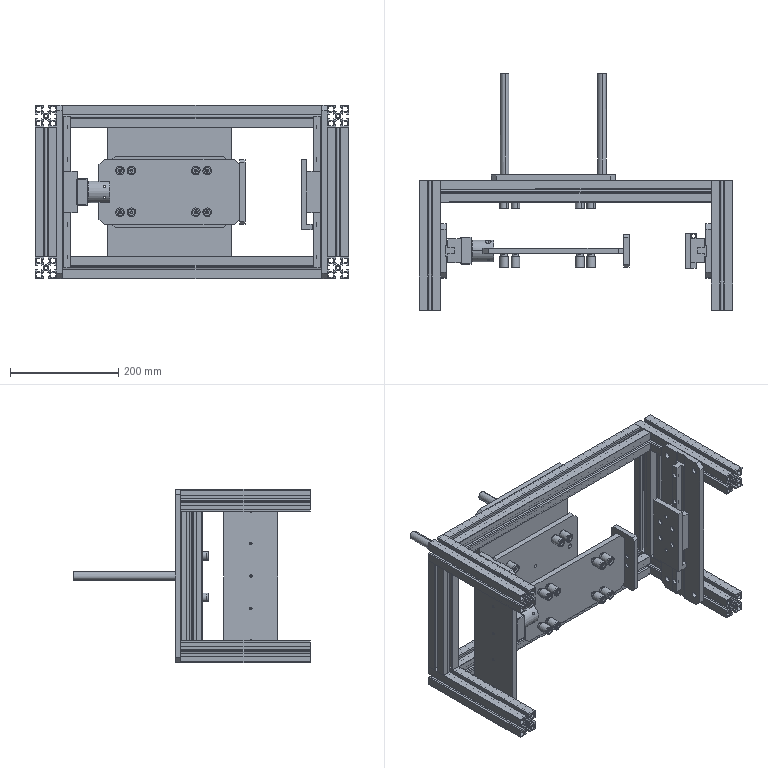Assembly | SolidWorks | mm | 41 component files | 41 solids | 1605 faces | box 580.04 x 437.8 x 320 mm | volume 3969042 mm3 | plane 981 | cylinder 594 | cone 30 | commonest cylinder face diameters 12 x96 5 x66 5.5 x44 16 x40 10 x40 4.2 x40 10.5 x40 5.3 x32
Bill of materials:
AdjustmentCylinderFixingPlate | 1 |  | Flat rectangular plate with four chamfered corners, one large central through-hole, and four small through-holes, one near each corner.
AdsorptionPlate | 1 |  | Thin, elongated rectangular plate with chamfered corners and eight through-holes in four pairs near the corners, plus two smaller holes near one short edge.
AdsorptionRelease | 1 |  | Thin rectangular plate with chamfered corners, eight larger through-holes in four pairs near the corners, and three smaller holes along the horizontal centerline (one at the center, one near each short edge).
AluminumProfile504 | 2 | 6061 Alloy | Long, straight prismatic extrusion with a square outer cross-section, an undercut slot centered on each of the four sides, hollow corner chambers, and a round central bore joined to the corners by diagonal webs.
Bearing6902 | 1 |  | Thick annular ring (flat washer- or spacer-like): a short hollow cylinder with a concentric through-bore and flat parallel faces.
GuideRailHGH-20CA-340 | 2 |  | Long, slender bar with a T-shaped cross-section (wide flange plus a narrower stem) and five evenly spaced small holes along its length.
GuideRod | 2 | AISI 304 | Long, straight, thick-walled round tube (hollow cylinder) with plain ends.
HGH20CASlider | 2 |  | Rectangular block with a full-height rectangular slot cut into one side, giving a C-shaped top profile, and four small holes in a rectangular pattern on one large face.
MainRotatingPlate | 1 |  | Moderately thick rectangular plate with chamfered corners and four small through-holes in a 2x2 pattern, placed off-center toward one long edge.
Profile240 | 6 | 6061 Alloy | Short length of square prismatic extrusion with an undercut slot on each side, hollow corner chambers, and a central round bore joined by diagonal webs.
RotationAxis | 1 |  | Cylindrical fork/clevis-like body: a large cylinder with a rectangular slot across one end that leaves two tines, cross-holes through the tines, and two stepped smaller-diameter coaxial bosses at the opposite end.
SidePlate | 2 |  | Elongated flat plate with chamfered corners, four corner holes, a centerline row of five small holes, and a stepped or recessed region on one face.
SlidingPlate | 1 |  | Square, fairly thick block with chamfered outer edges, a large central through bore, and four smaller through holes, one near each corner.
SwingCylinderMountingPlate | 1 |  | L-shaped bracket: a tall rectangular plate with a short perpendicular foot along its bottom edge. The plate has six through holes and the foot has one larger hole.
SuctionPositioning | 16 | AISI 304 | Stepped hollow cylinder: a larger-diameter section and a smaller-diameter section on one axis, with an axial bore all the way through and one radial cross hole through the smaller section.
UpperAndLowerCylinderMountingPlate | 1 |  | Thin, flat rectangular plate with chamfered corners. It has four elongated slots, one large central hole, two smaller holes to either side, and small holes clustered around each of these three holes.
Mates:
1. coincident | assembly face at (2922.223, 3603.91, 956.241) dir (0.0001552, -1, 0) | assembly face at (1637.199, 3603.71, 939.241) dir (-0.0001552, 1, 0)
2. distance | assembly face at (2922.22, 3618.61, 959.241) dir (0, 0, 1) | assembly face at (1502.198, 3608.689, 999.241) dir (0, 0, -1)
3. coincident | assembly face at (-641.795, 3680.91, 1199.241) dir (0, 0, -1) | assembly face at (1579.721, 3703.352, 1199.241) dir (0, 0, 1)
4. concentric | assembly face at (1554.723, 3703.361, 1192.741) dir (0, 0, -1) r 5.5 | assembly face at (1554.723, 3703.361, 965.741) dir (0, 0, 1) r 5.5
5. coincident | assembly face at (2922.211, 3680.91, 959.241) dir (0, 0, 1) | assembly face at (1529.723, 3703.357, 959.241) dir (0, 0, -1)
6. width | AdsorptionPlate-1 face at (1702.163, 3838.72, 1079.241) dir (-0.0001552, 1, 0) | AdsorptionPlate-1 face at (1702.164, 3828.72, 1079.241) dir (0.0001552, -1, 0) | MainRotatingPlate-1 face at (1832.159, 3863.74, 1019.241) dir (-0.0001552, 1, 0) | MainRotatingPlate-1 face at (1832.168, 3803.74, 1019.241) dir (0.0001552, -1, 0)
7. coincident | MainRotatingPlate-1 face at (1832.163, 3833.74, 1079.241) dir (-1, -0.0001552, 0) | AdsorptionPlate-1 face at (1832.163, 3838.74, 1011.741) dir (1, 0.0001552, 0)
8. width | AdsorptionPlate-1 face at (1832.163, 3838.74, 1019.241) dir (0, 0, -1) | AdsorptionPlate-1 face at (1832.163, 3838.74, 1139.241) dir (0, 0, 1) | MainRotatingPlate-1 face at (1832.159, 3863.74, 1139.241) dir (0, 0, 1) | MainRotatingPlate-1 face at (1832.159, 3863.74, 1019.241) dir (0, 0, -1)
9. coincident | AdsorptionPlate-1 face at (1702.163, 3838.72, 1079.241) dir (-0.0001552, 1, 0) | UltrasonicProductSuction-1/SuctionPositioning-1 face at (1772.163, 3838.731, 1041.741) dir (-0.0001552, 1, 0)
10. concentric | AdsorptionPlate-1 face at (1772.163, 3838.731, 1041.741) dir (-0.0001552, 1, 0) r 6 | UltrasonicProductSuction-1/SuctionPositioning-1 face at (1772.166, 3813.731, 1041.741) dir (-0.0001552, 1, 0) r 6
11. concentric | AdsorptionPlate-1 face at (1751.163, 3838.728, 1041.741) dir (-0.0001552, 1, 0) r 6 | UltrasonicProductSuction-9/SuctionPositioning-1 face at (1751.166, 3813.728, 1041.741) dir (-0.0001552, 1, 0) r 6
12. coincident | UltrasonicProductSuction-1/SuctionPositioning-1 face at (1772.168, 3803.731, 1041.741) dir (0.0001552, -1, 0) | UltrasonicProductSuction-9/SuctionPositioning-1 face at (1751.168, 3803.728, 1041.741) dir (0.0001552, -1, 0)
13. coincident | AdsorptionPlate-1 face at (1572.163, 3838.7, 1011.741) dir (-1, -0.0001552, 0) | RotationAxis-1 face at (1572.163, 3833.7, 1079.241) dir (1, 0.0001552, 0)
14. concentric | GuideRod-1 face at (1792.112, 4161.484, 1079.241) dir (0.0001552, -1, 0) r 8 | AdsorptionRelease-1 face at (1792.147, 3936.484, 1079.241) dir (-0.0001552, 1, 0) r 8
15. coincident | GuideRod-1 face at (1792.147, 3936.484, 1079.241) dir (0.0001552, -1, 0) | AdsorptionRelease-1 face at (1792.147, 3936.484, 1079.241) dir (-0.0001552, 1, 0)
16. concentric | AdsorptionRelease-1 face at (1772.147, 3941.481, 1039.741) dir (-0.0001552, 1, 0) r 6 | UltrasonicProductSuction-17/SuctionPositioning-1 face at (1772.15, 3921.481, 1039.741) dir (-0.0001552, 1, 0) r 6
17. coincident | AdsorptionRelease-1 face at (1702.148, 3931.47, 1079.241) dir (0.0001552, -1, 0) | UltrasonicProductSuction-17/SuctionPositioning-1 face at (1772.148, 3931.481, 1039.741) dir (-0.0001552, 1, 0)
18. concentric | AdsorptionRelease-1 face at (1751.147, 3941.478, 1039.741) dir (-0.0001552, 1, 0) r 6 | UltrasonicProductSuction-22/SuctionPositioning-1 face at (1751.15, 3921.478, 1039.741) dir (-0.0001552, 1, 0) r 6
19. coincident | UltrasonicProductSuction-17/SuctionPositioning-1 face at (1772.151, 3911.481, 1039.741) dir (0.0001552, -1, 0) | UltrasonicProductSuction-22/SuctionPositioning-1 face at (1751.151, 3911.478, 1039.741) dir (0.0001552, -1, 0)
20. width | SidePlate-1 face at (1504.156, 3883.689, 919.241) dir (-0.0001552, 1, 0) | SidePlate-1 face at (1504.171, 3783.689, 919.241) dir (0.0001552, -1, 0) | RotationAxis-1 face at (1552.163, 3833.697, 1079.241) dir (1, 0.0001552, 0) r 20
21. coincident | GuideRailHGH-20CA-340-1 face at (1506.762, 3839.19, 925.579) dir (-0.0001552, 1, 0) | HGH20CASlider-1 face at (1506.762, 3839.19, 1023.538) dir (0.0001552, -1, 0)
22. coincident | GuideRailHGH-20CA-340-1 face at (1519.665, 3823.692, 1219.241) dir (1, 0.0001552, 0) | HGH20CASlider-1 face at (1519.662, 3839.192, 1023.538) dir (-1, -0.0001552, 0)
23. width | SidePlate-1 face at (1504.156, 3883.689, 919.241) dir (-0.0001552, 1, 0) | SidePlate-1 face at (1504.171, 3783.689, 919.241) dir (0.0001552, -1, 0) | GuideRailHGH-20CA-340-1 face at (1506.764, 3828.19, 925.579) dir (0.0001552, -1, 0) | GuideRailHGH-20CA-340-1 face at (1506.762, 3839.19, 925.579) dir (-0.0001552, 1, 0)
24. width | GuideRailHGH-20CA-340-1 face at (1510.913, 3833.691, 939.241) dir (0, 0, -1) | GuideRailHGH-20CA-340-1 face at (1510.913, 3833.691, 1219.241) dir (0, 0, 1) | SidePlate-1 face at (1504.171, 3783.689, 1239.241) dir (0, 0, 1) | SidePlate-1 face at (1504.171, 3783.689, 919.241) dir (0, 0, -1)
25. concentric | RotationAxis-1 face at (1542.163, 3833.695, 1079.241) dir (1, 0.0001552, 0) r 7.5 | Bearing6902-1 face at (1548.163, 3833.696, 1079.241) dir (-1, -0.0001552, 0) r 7.5
26. coincident | RotationAxis-1 face at (1548.163, 3833.696, 1079.241) dir (-1, -0.0001552, 0) | Bearing6902-1 face at (1548.163, 3833.696, 1079.241) dir (1, 0.0001552, 0)
27. coincident | Bearing6902-1 face at (1541.163, 3833.695, 1079.241) dir (-1, -0.0001552, 0) | SlidingPlate-1 face at (1541.163, 3833.695, 1079.241) dir (1, 0.0001552, 0)
28. concentric | Bearing6902-1 face at (1548.163, 3833.696, 1079.241) dir (-1, -0.0001552, 0) r 14 | SlidingPlate-1 face at (1541.163, 3833.695, 1079.241) dir (1, 0.0001552, 0) r 14
29. concentric | HGH20CASlider-1 face at (1532.161, 3849.694, 1061.241) dir (1, 0.0001552, 0) r 2.1 | SlidingPlate-1 face at (1551.161, 3849.697, 1061.241) dir (1, 0.0001552, 0) r 5
30. concentric | HGH20CASlider-2 face at (1956.166, 3817.76, 1061.241) dir (-1, -0.0001552, 0) r 2.1 | SwingCylinderMountingPlate-1 face at (1946.166, 3817.758, 1061.241) dir (-1, -0.0001552, 0) r 2.75
31. concentric | HGH20CASlider-2 face at (1956.161, 3849.76, 1097.241) dir (-1, -0.0001552, 0) r 2.1 | SwingCylinderMountingPlate-1 face at (1946.161, 3849.758, 1097.241) dir (-1, -0.0001552, 0) r 2.75
32. coincident | HGH20CASlider-2 face at (1956.163, 3833.76, 1079.241) dir (-1, -0.0001552, 0) | SwingCylinderMountingPlate-1 face at (1956.163, 3833.76, 1079.241) dir (1, 0.0001552, 0)
33. coincident | GuideRailHGH-20CA-340-2 face at (1981.562, 3839.264, 1232.903) dir (-0.0001552, 1, 0) | HGH20CASlider-2 face at (1981.562, 3839.264, 1134.944) dir (0.0001552, -1, 0)
34. coincident | GuideRailHGH-20CA-340-2 face at (1968.665, 3823.762, 939.241) dir (-1, -0.0001552, 0) | HGH20CASlider-2 face at (1968.662, 3839.262, 1134.944) dir (1, 0.0001552, 0)
35. coincident | GuideRailHGH-20CA-340-1 face at (1510.913, 3833.691, 939.241) dir (0, 0, -1) | GuideRailHGH-20CA-340-2 face at (1977.413, 3833.763, 939.241) dir (0, 0, -1)
36. coincident | Profile240-4 face at (2033.926, 5363.772, 959.241) dir (1, 0.0001552, 0) | Profile240-5 face at (2033.926, 5363.772, 1239.241) dir (1, 0.0001552, 0)
37. coincident | Profile240-4 face at (2096.808, 3963.781, 919.241) dir (-0.0001552, 1, 0) | Profile240-5 face at (2096.808, 3963.781, 1199.241) dir (-0.0001552, 1, 0)
38. coincident | Profile240-4 face at (2096.808, 3963.781, 919.241) dir (-0.0001552, 1, 0) | Profile240-6 face at (1556.808, 3963.698, 919.241) dir (-0.0001552, 1, 0)
39. coincident | Profile240-4 face at (1993.926, 5363.766, 919.241) dir (0, 0, -1) | Profile240-6 face at (1453.926, 5363.682, 919.241) dir (0, 0, -1)
40. coincident | SidePlate-1 face at (1494.163, 3833.688, 1079.241) dir (-1, -0.0001552, 0) | Profile240-6 face at (1493.926, 5363.688, 959.241) dir (1, 0.0001552, 0)
41. coincident | Profile240-6 face at (1493.926, 5363.688, 959.241) dir (1, 0.0001552, 0) | Profile240-7 face at (1493.926, 5363.688, 1239.241) dir (1, 0.0001552, 0)
42. coincident | Profile240-6 face at (1556.808, 3963.698, 919.241) dir (-0.0001552, 1, 0) | Profile240-7 face at (1556.808, 3963.698, 1199.241) dir (-0.0001552, 1, 0)
43. coincident | Profile240-5 face at (1993.926, 5363.766, 1239.241) dir (0, 0, 1) | Profile240-7 face at (1453.926, 5363.682, 1239.241) dir (0, 0, 1)
44. coincident | Profile240-5 face at (1993.926, 5363.766, 1199.241) dir (0, 0, -1) | Profile240-8 face at (2096.808, 3963.781, 1199.241) dir (0, 0, 1)
45. coincident | Profile240-5 face at (2096.808, 3963.781, 1199.241) dir (-0.0001552, 1, 0) | Profile240-8 face at (1994.143, 3963.766, 2599.241) dir (-0.0001552, 1, 0)
46. coincident | Profile240-5 face at (2033.926, 5363.772, 1239.241) dir (1, 0.0001552, 0) | Profile240-8 face at (2034.149, 3923.772, 2599.241) dir (1, 0.0001552, 0)
47. coincident | Profile240-7 face at (1493.926, 5363.688, 1239.241) dir (1, 0.0001552, 0) | Profile240-9 face at (1494.149, 3923.688, 2599.241) dir (1, 0.0001552, 0)
48. coincident | Profile240-7 face at (1453.926, 5363.682, 1199.241) dir (0, 0, -1) | Profile240-9 face at (1556.808, 3963.698, 1199.241) dir (0, 0, 1)
49. coincident | Profile240-7 face at (1556.808, 3963.698, 1199.241) dir (-0.0001552, 1, 0) | Profile240-9 face at (1454.143, 3963.682, 2599.241) dir (-0.0001552, 1, 0)
50. coincident | Profile240-4 face at (2096.808, 3963.781, 919.241) dir (-0.0001552, 1, 0) | AluminumProfile504-1 face at (354.143, 3963.511, 919.241) dir (-0.0001552, 1, 0)
51. coincident | Profile240-4 face at (1993.926, 5363.766, 919.241) dir (0, 0, -1) | AluminumProfile504-1 face at (354.143, 3963.511, 919.241) dir (0, 0, -1)
52. coincident | Profile240-6 face at (1493.926, 5363.688, 959.241) dir (1, 0.0001552, 0) | AluminumProfile504-1 face at (1494.159, 3861.023, 959.241) dir (-1, -0.0001552, 0)
53. coincident | Profile240-5 face at (2096.808, 3963.781, 1199.241) dir (-0.0001552, 1, 0) | AluminumProfile504-2 face at (354.143, 3963.511, 1199.241) dir (-0.0001552, 1, 0)
54. coincident | Profile240-5 face at (1993.926, 5363.766, 1239.241) dir (0, 0, 1) | AluminumProfile504-2 face at (354.149, 3923.511, 1239.241) dir (0, 0, 1)
55. coincident | Profile240-5 face at (1993.926, 5363.766, 1239.241) dir (-1, -0.0001552, 0) | AluminumProfile504-2 face at (1994.143, 3963.766, 1199.241) dir (1, 0.0001552, 0)
56. concentric | UpperAndLowerCylinderMountingPlate-1 face at (1714.642, 3968.722, 1109.241) dir (-0.0001552, 1, 0) r 1.65 | AdjustmentCylinderFixingPlate-1 face at (1714.642, 3973.722, 1109.241) dir (-0.0001552, 1, 0) r 2.15
57. concentric | UpperAndLowerCylinderMountingPlate-1 face at (1689.642, 3968.718, 1049.241) dir (-0.0001552, 1, 0) r 1.65 | AdjustmentCylinderFixingPlate-1 face at (1689.642, 3973.718, 1049.241) dir (-0.0001552, 1, 0) r 2.15
58. coincident | UpperAndLowerCylinderMountingPlate-1 face at (1702.142, 3968.72, 1079.241) dir (-0.0001552, 1, 0) | AdjustmentCylinderFixingPlate-1 face at (1702.142, 3968.72, 1079.241) dir (0.0001552, -1, 0)
59. coincident | SidePlate-2 face at (1994.163, 3833.766, 1079.241) dir (1, 0.0001552, 0) | Profile240-4 face at (1993.926, 5363.766, 959.241) dir (-1, -0.0001552, 0)
60. concentric | GuideRailHGH-20CA-340-2 face at (1968.663, 3833.762, 959.241) dir (-1, -0.0001552, 0) r 5 | SidePlate-2 face at (1984.163, 3833.764, 959.241) dir (-1, -0.0001552, 0) r 2.1
61. coincident | SidePlate-1 face at (1504.171, 3783.689, 919.241) dir (0, 0, -1) | SidePlate-2 face at (1984.156, 3883.764, 919.241) dir (0, 0, -1)
62. coincident | Profile240-7 face at (1493.926, 5363.688, 1239.241) dir (1, 0.0001552, 0) | AluminumProfile504-2 face at (1494.143, 3963.688, 1301.906) dir (-1, -0.0001552, 0)
63. coincident | GuideRailHGH-20CA-340-2 face at (1986.165, 3823.764, 939.241) dir (1, 0.0001552, 0) | SidePlate-2 face at (1986.163, 3833.764, 1079.241) dir (-1, -0.0001552, 0)
64. concentric | FlipSupportMechanism face at (184.908, -113.55, 372) dir (0, 0, -1) r 8 | FlipSupportMechanism face at (184.908, -113.55, 377) dir (0, 0, -1) r 8
65. concentric | SynchronousBeltDrive1 face at (205.548, 24.293, 3390) dir (0, 0, 1) r 5.25 | SynchronousBeltDrive1 face at (205.548, 24.293, 1118) dir (0, 0, -1) r 7.5
66. concentric | SynchronousBeltDrive1 face at (205.548, -15.707, 3390) dir (0, 0, 1) r 5.25 | SynchronousBeltDrive1 face at (205.548, -15.707, 1118) dir (0, 0, -1) r 7.5
67. coincident | SynchronousBeltDrive1 face at (188.548, -32.707, 1130) dir (0, 0, -1) | SynchronousBeltDrive1 face at (205.548, 4.293, 1130) dir (0, 0, 1)
68. concentric | SynchronousBeltDrive1 face at (205.548, 24.293, 3390) dir (0, 0, 1) r 5.25 | SynchronousBeltDrive1 face at (205.548, 24.293, 3402) dir (0, 0, 1) r 7.5
69. concentric | SynchronousBeltDrive1 face at (205.548, -15.707, 3390) dir (0, 0, 1) r 5.25 | SynchronousBeltDrive1 face at (205.548, -15.707, 3402) dir (0, 0, 1) r 7.5
70. coincident | SynchronousBeltDrive1 face at (205.548, 4.293, 3390) dir (0, 0, 1) | SynchronousBeltDrive1 face at (205.548, 4.293, 3390) dir (0, 0, -1)
71. concentric | SynchronousBeltDrive1 axis at (225.548, 25.293, 1107) dir (-1, 0, 0) | SynchronousBeltDrive1 face at (221.548, 25.293, 1107) dir (1, 0, 0) r 5.5
72. concentric | SynchronousBeltDrive1 axis at (150.545, -6.707, 1107) dir (-1, 0, 0) | SynchronousBeltDrive1 face at (146.545, -6.707, 1107) dir (1, 0, 0) r 5.5
73. coincident | SynchronousBeltDrive1 face at (215.548, 44.293, 1096) dir (-1, 0, 0) | SynchronousBeltDrive1 face at (215.548, -14.207, 1118) dir (1, 0, 0)
74. concentric | SynchronousBeltDrive1 axis at (225.548, -16.707, 3413) dir (-1, 0, 0) | SynchronousBeltDrive1 face at (221.548, -16.707, 3413) dir (1, 0, 0) r 5.5
75. concentric | SynchronousBeltDrive1 axis at (150.545, 15.293, 3413) dir (-1, 0, 0) | SynchronousBeltDrive1 face at (146.545, 15.293, 3413) dir (1, 0, 0) r 5.5
76. coincident | SynchronousBeltDrive1 face at (215.548, -35.707, 3424) dir (-1, 0, 0) | SynchronousBeltDrive1 face at (215.548, 22.793, 3402) dir (1, 0, 0)
77. concentric | SynchronousBeltDrive1 face at (205.548, -15.707, 3390) dir (0, 0, 1) r 5.25 | SynchronousBeltDrive1 face at (205.548, -15.707, 3402) dir (0, 0, 1) r 7.5
78. concentric | SynchronousBeltDrive1 face at (205.548, 24.293, 3390) dir (0, 0, 1) r 5.25 | SynchronousBeltDrive1 face at (205.548, 24.293, 3402) dir (0, 0, 1) r 7.5
79. coincident | SynchronousBeltDrive1 face at (205.548, 4.293, 3390) dir (0, 0, 1) | SynchronousBeltDrive1 face at (205.548, 4.293, 3390) dir (0, 0, -1)
80. concentric | SynchronousBeltDrive1 face at (225.548, -14.067, 3429) dir (-1, 0, 0) r 5.5 | SynchronousBeltDrive1 face at (221.548, -14.067, 3429) dir (1, 0, 0) r 5.5
81. concentric | SynchronousBeltDrive1 face at (225.548, 7.933, 3429) dir (-1, 0, 0) r 5.5 | SynchronousBeltDrive1 face at (221.548, 7.933, 3429) dir (1, 0, 0) r 5.5
82. coincident | SynchronousBeltDrive1 face at (215.548, -35.707, 3438) dir (-1, 0, 0) | SynchronousBeltDrive1 face at (215.548, 25.433, 3418) dir (1, 0, 0)
83. concentric | SynchronousBeltDrive1 face at (205.548, -15.707, 3390) dir (0, 0, 1) r 5.25 | SynchronousBeltDrive1 face at (205.548, -15.707, 818) dir (0, 0, -1) r 7.5
84. concentric | SynchronousBeltDrive1 face at (205.548, 24.293, 3390) dir (0, 0, 1) r 5.25 | SynchronousBeltDrive1 face at (205.548, 24.293, 818) dir (0, 0, -1) r 7.5
85. coincident | SynchronousBeltDrive1 face at (188.548, -32.707, 830) dir (0, 0, -1) | SynchronousBeltDrive1 face at (165.548, 4.293, 830) dir (0, 0, 1)
86. distance | SynchronousBeltDrive1 face at (365.548, 4.293, 3510) dir (0, 0, 1) | SynchronousBeltDrive1 face at (205.548, 4.293, 3390) dir (0, 0, -1)
87. coincident | SynchronousBeltDrive1 face at (348.548, -32.707, 710) dir (0, 0, -1) | SynchronousBeltDrive1 face at (348.548, 44.293, 710) dir (0, 0, -1)
88. coincident | SynchronousBeltDrive1 face at (382.548, 44.293, 3510) dir (0, 1, 0) | SynchronousBeltDrive1 face at (365.548, 44.293, 750) dir (0, -1, 0)
89. coincident | SynchronousBeltDrive1 face at (385.548, -10.407, 3510) dir (1, 0, 0) | SynchronousBeltDrive1 face at (385.548, 44.293, 735.3) dir (1, 0, 0)
90. coincident | SynchronousBeltDrive1 face at (360.248, 44.293, 3510) dir (0, 1, 0) | SynchronousBeltDrive1 face at (365.548, 44.293, 3470) dir (0, -1, 0)
91. coincident | SynchronousBeltDrive1 face at (365.548, 4.293, 3510) dir (0, 0, 1) | SynchronousBeltDrive1 face at (360.248, 44.293, 3510) dir (0, 0, 1)
92. coincident | SynchronousBeltDrive1 face at (385.548, -10.407, 3510) dir (1, 0, 0) | SynchronousBeltDrive1 face at (385.548, 44.293, 3455.3) dir (1, 0, 0)